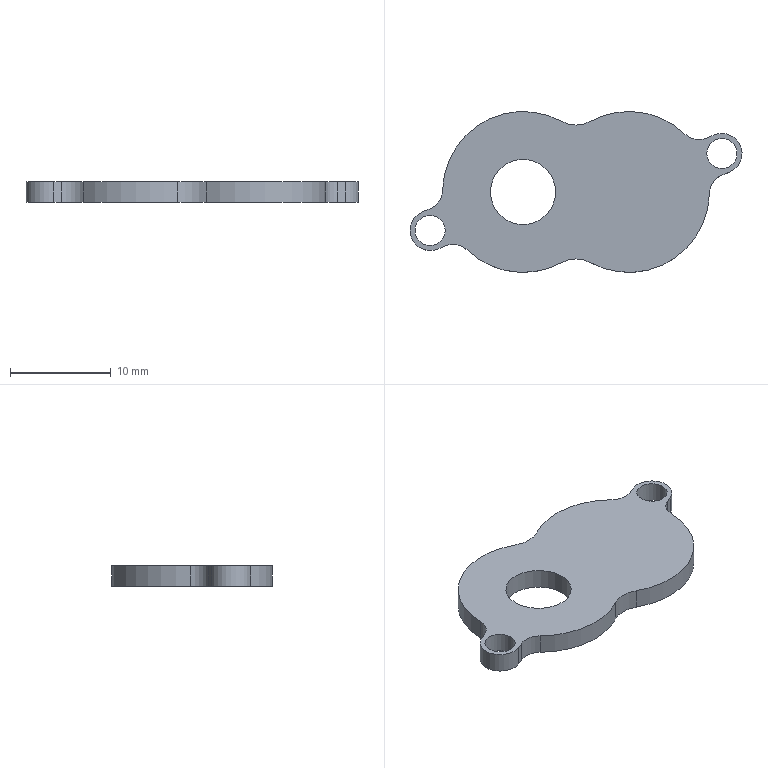Component | NX | DRIVE_END_SMALL_COVER | 1 solid | 21 faces | volume 682 mm3 | cylinder 15 | plane 6 | commonest cylinder face diameters 4 x6 16 x4 6 x2 3 x2 6.5 x1